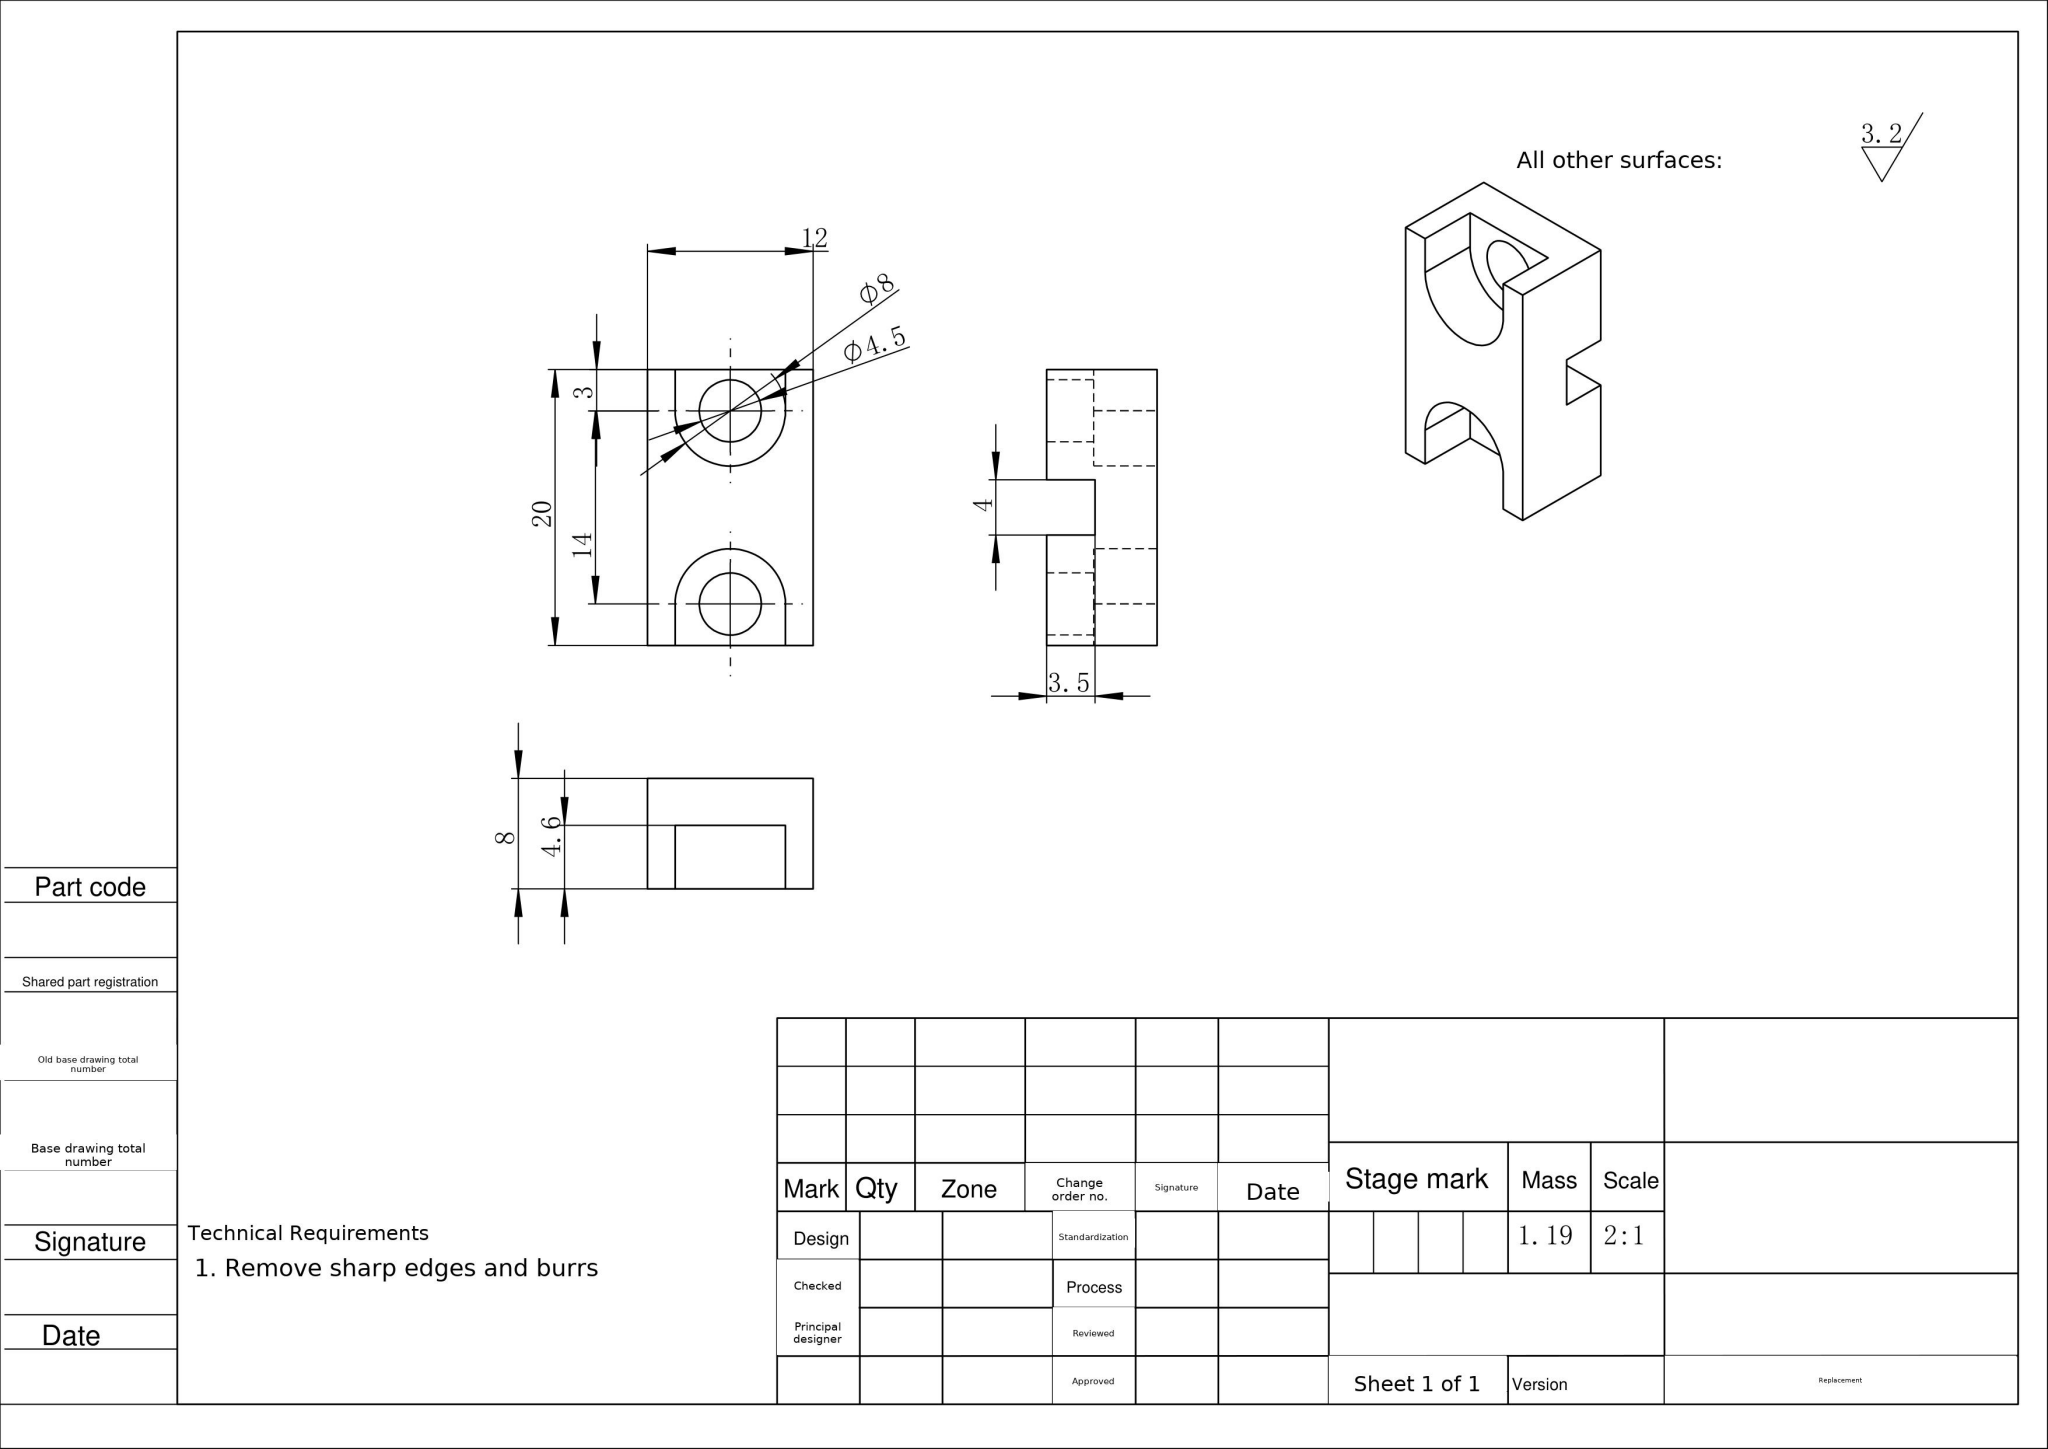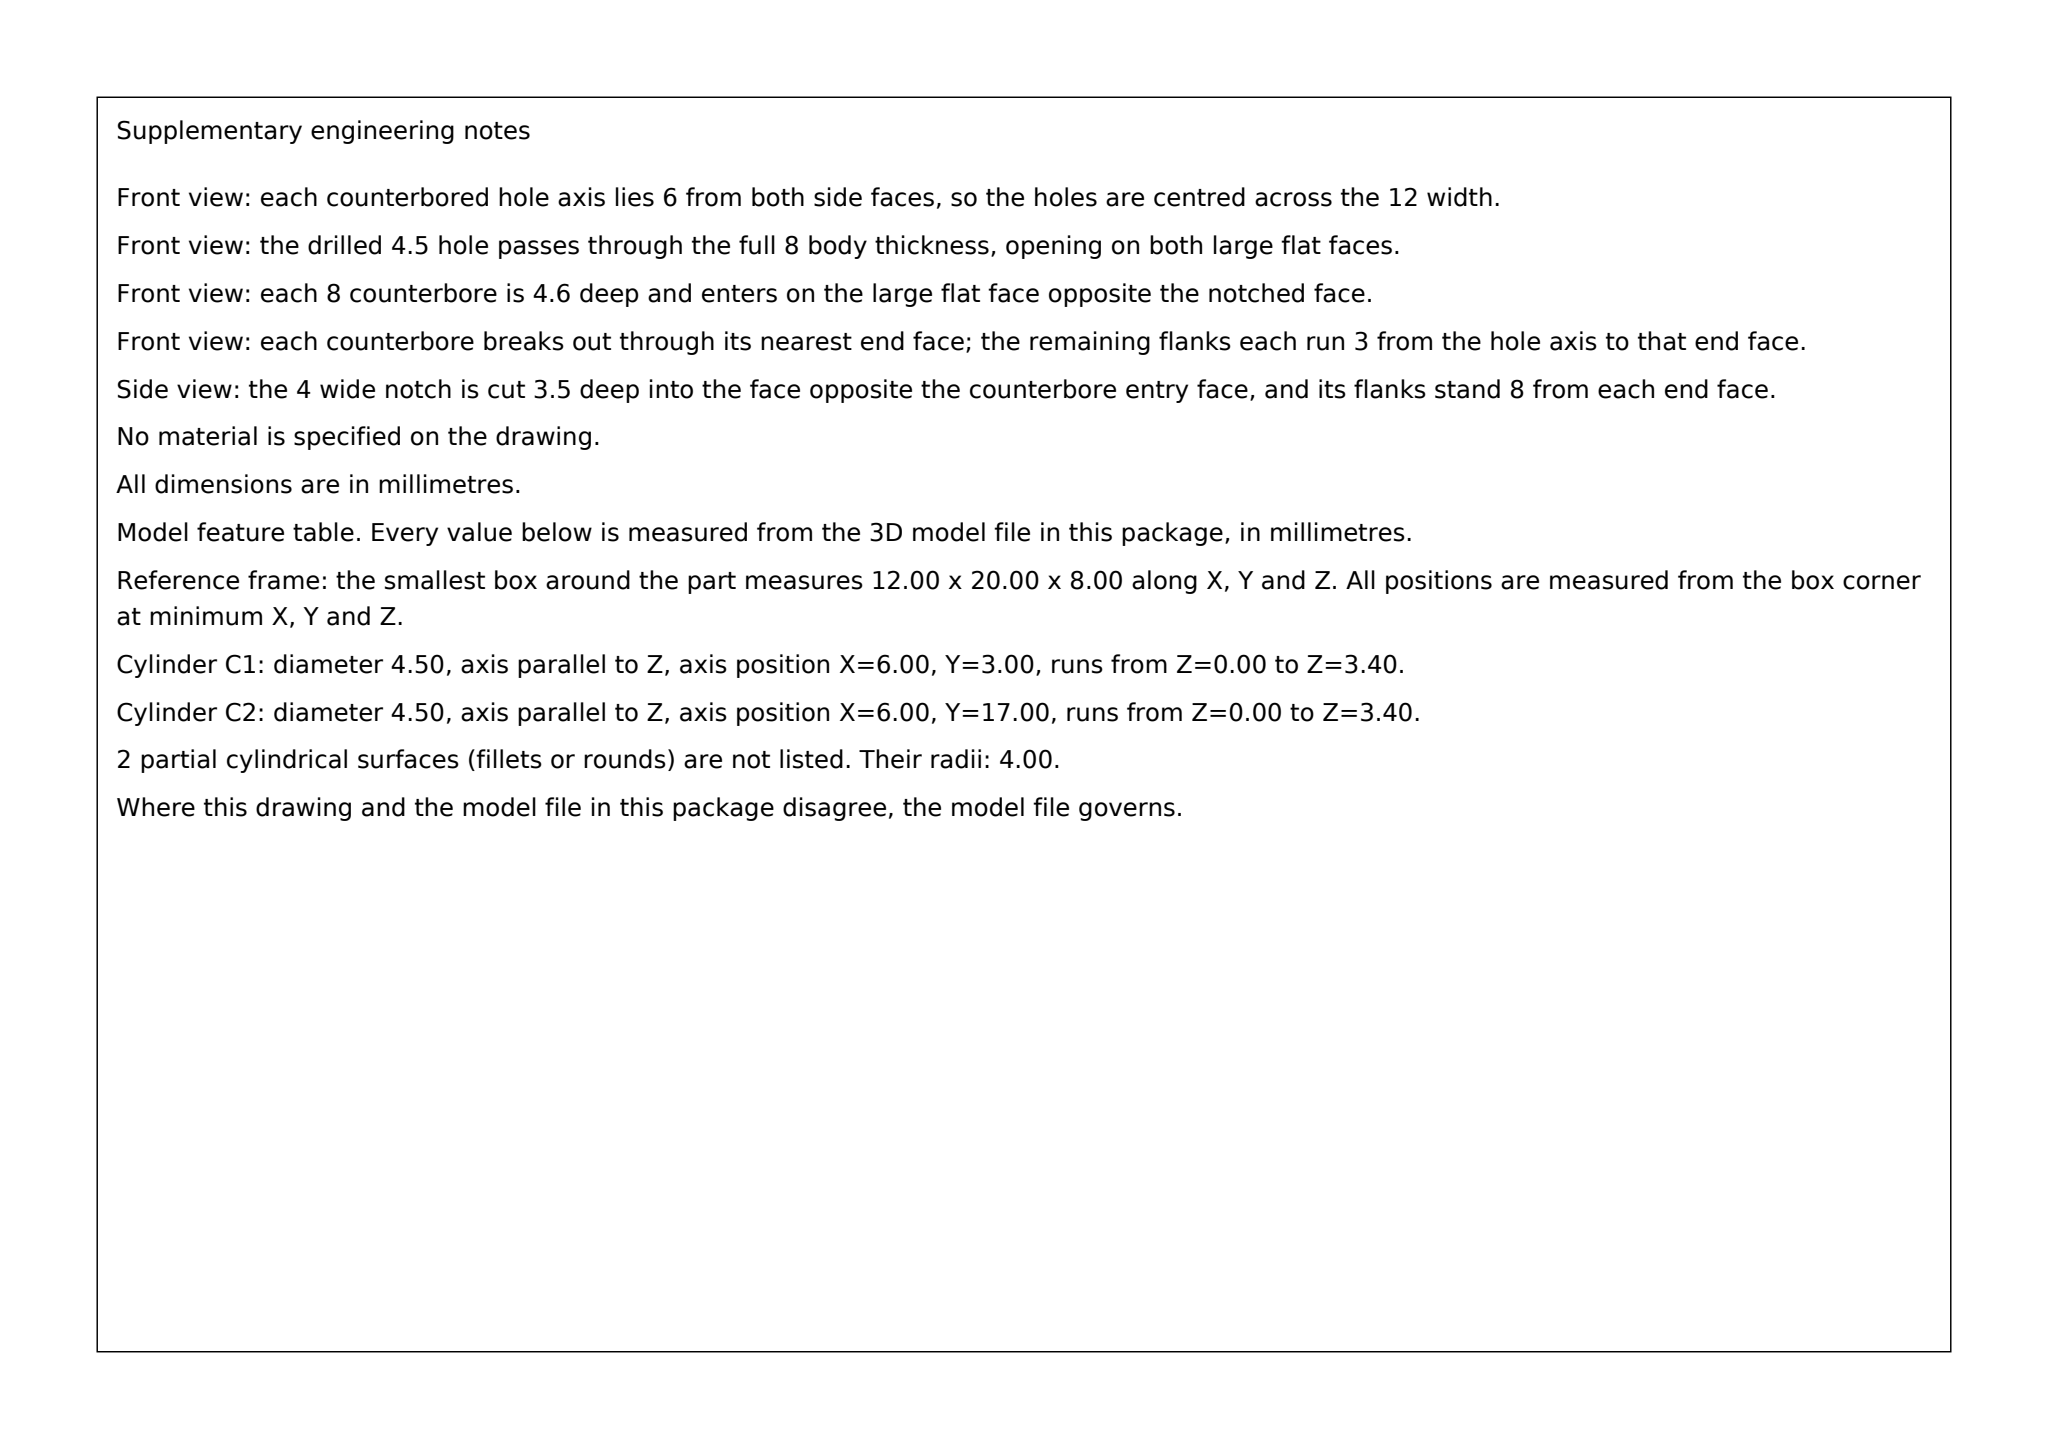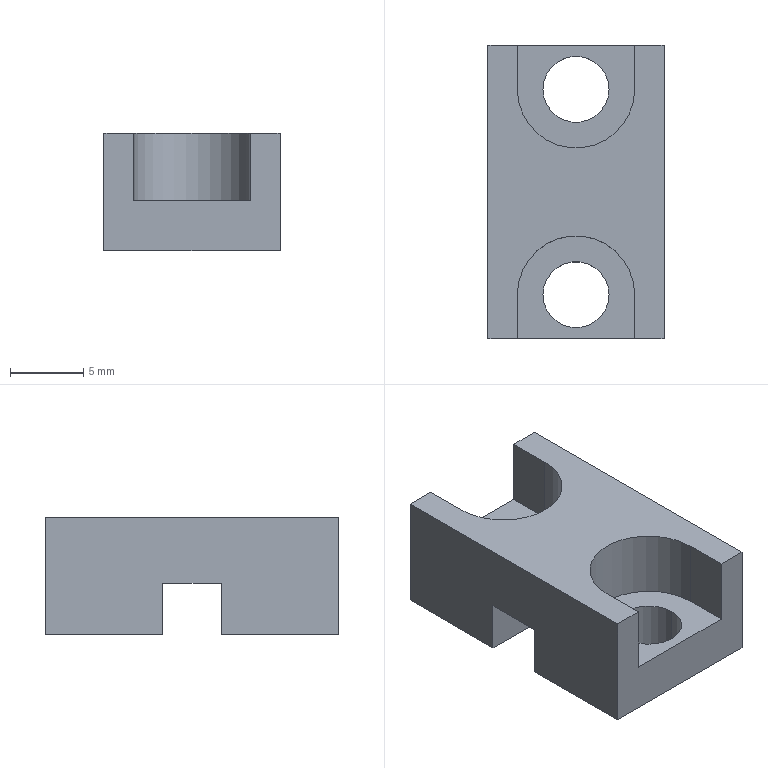Part | SolidWorks | mm | 1 solid | 22 faces | box 12 x 20 x 8 mm | volume 1192 mm3 | plane 16 | cylinder 6 | commonest cylinder face diameters 4.5 x4 8 x2
Drawing notes:
4 WIDE GROOVE SYM ABOUT 20 CL (8 FROM EACH END) | from the solid: y-planes at 8.0 and 12.0 within 0-20 bbox: 4 wide, centered on y=10
GROOVE THRU FULL 12 WIDTH, 3.5 DEEP | from the solid: groove faces span x=0 to 12 (bbox x=12); z-plane at 3.5 gives depth
build123d program:
from build123d import *

# Parameters (mm, degrees)
SKETCH1_W                                            = 12
SKETCH1_H                                            = 20
BOSS_EXTRUDE1_DEPTH                                  = 8
SKETCH2_W                                            = 12
SKETCH2_H                                            = 4
CUT_EXTRUDE1_DEPTH                                   = 3.5
HOLE_SIZE_ACCORDING_TO_TYPE_1_OF_HEXAGON_D           = 4.5
HOLE_SIZE_ACCORDING_TO_TYPE_1_OF_HEXAGON_DEPTH       = 11.5
HOLE_SIZE_ACCORDING_TO_TYPE_1_OF_HEXAGON_CBORE_D     = 8
HOLE_SIZE_ACCORDING_TO_TYPE_1_OF_HEXAGON_CBORE_DEPTH = 4.6
HOLE_SIZE_ACCORDING_TO_TYPE_1_OF_HEXAGON_TIP         = 1.352
SKETCH5_W                                            = 8
SKETCH5_H                                            = 8.409
SKETCH5_H_2                                          = 4.715
CUT_EXTRUDE2_DEPTH                                   = 4.6


with BuildPart() as part:
    # Sketch1 → Boss-Extrude1 (new body)
    with BuildSketch(Plane.XY):
        with Locations((-273.963, 122.5)):
            Rectangle(SKETCH1_W, SKETCH1_H)
    extrude(amount=BOSS_EXTRUDE1_DEPTH)

    # Sketch2 → Cut-Extrude1 (cut)
    with BuildSketch(Plane(origin=(0, 0, 0), x_dir=(-1, 0, 0), z_dir=(0, 0, -1))):
        with Locations((273.963, 122.5)):
            Rectangle(SKETCH2_W, SKETCH2_H)
    extrude(amount=-CUT_EXTRUDE1_DEPTH, mode=Mode.SUBTRACT)

    # Hole Size_According to_Type 1 of Hexagon
    with Locations(Plane.XY.offset(8)):
        with Locations((-273.963, 129.5), (-273.963, 115.5)):
            CounterBoreHole(HOLE_SIZE_ACCORDING_TO_TYPE_1_OF_HEXAGON_D / 2, HOLE_SIZE_ACCORDING_TO_TYPE_1_OF_HEXAGON_CBORE_D / 2, HOLE_SIZE_ACCORDING_TO_TYPE_1_OF_HEXAGON_CBORE_DEPTH, depth=HOLE_SIZE_ACCORDING_TO_TYPE_1_OF_HEXAGON_DEPTH)
            with Locations((0, 0, -(HOLE_SIZE_ACCORDING_TO_TYPE_1_OF_HEXAGON_DEPTH + HOLE_SIZE_ACCORDING_TO_TYPE_1_OF_HEXAGON_TIP / 2))):  # 118° drill point
                Cone(0, HOLE_SIZE_ACCORDING_TO_TYPE_1_OF_HEXAGON_D / 2, HOLE_SIZE_ACCORDING_TO_TYPE_1_OF_HEXAGON_TIP, mode=Mode.SUBTRACT)

    # Sketch5 → Cut-Extrude2 (cut)
    with BuildSketch(Plane.XY.offset(8)):
        with Locations((-273.963, 133.705)):
            Rectangle(SKETCH5_W, SKETCH5_H)
        with Locations((-273.963, 113.143)):
            Rectangle(SKETCH5_W, SKETCH5_H_2)
    extrude(amount=-CUT_EXTRUDE2_DEPTH, mode=Mode.SUBTRACT)


solid = part.part
STEP:
#1=CARTESIAN_POINT('',(-271.713,129.5,0.));
#2=VERTEX_POINT('',#1);
#3=CARTESIAN_POINT('',(-276.213,129.5,0.));
#4=VERTEX_POINT('',#3);
#5=CARTESIAN_POINT('',(-273.963,129.5,0.));
#6=DIRECTION('',(0.,0.,-1.));
#7=DIRECTION('',(-1.,0.,0.));
#8=AXIS2_PLACEMENT_3D('',#5,#6,#7);
#9=CIRCLE('',#8,2.25);
#10=EDGE_CURVE('',#2,#4,#9,.T.);
#11=ORIENTED_EDGE('',*,*,#10,.T.);
#12=CARTESIAN_POINT('',(-276.213,129.5,3.4));
#13=VERTEX_POINT('',#12);
#14=CARTESIAN_POINT('',(-276.213,129.5,8.));
#15=DIRECTION('',(0.,0.,1.));
#16=VECTOR('',#15,1000.);
#17=LINE('',#14,#16);
#18=EDGE_CURVE('',#4,#13,#17,.T.);
#19=ORIENTED_EDGE('',*,*,#18,.T.);
#20=CARTESIAN_POINT('',(-271.713,129.5,3.4));
#21=VERTEX_POINT('',#20);
#22=CARTESIAN_POINT('',(-273.963,129.5,3.4));
#23=DIRECTION('',(0.,0.,1.));
#24=DIRECTION('',(1.,0.,0.));
#25=AXIS2_PLACEMENT_3D('',#22,#23,#24);
#26=CIRCLE('',#25,2.25);
#27=EDGE_CURVE('',#13,#21,#26,.T.);
#28=ORIENTED_EDGE('',*,*,#27,.T.);
#29=CARTESIAN_POINT('',(-271.713,129.5,8.));
#30=DIRECTION('',(0.,0.,1.));
#31=VECTOR('',#30,1000.);
#32=LINE('',#29,#31);
#33=EDGE_CURVE('',#2,#21,#32,.T.);
#34=ORIENTED_EDGE('',*,*,#33,.F.);
#35=EDGE_LOOP('',(#11,#19,#28,#34));
#36=FACE_OUTER_BOUND('',#35,.T.);
#37=CARTESIAN_POINT('',(-273.963,129.5,8.));
#38=DIRECTION('',(0.,0.,1.));
#39=DIRECTION('',(1.,0.,0.));
#40=AXIS2_PLACEMENT_3D('',#37,#38,#39);
#41=CYLINDRICAL_SURFACE('',#40,2.25);
#42=ADVANCED_FACE('',(#36),#41,.F.);
#43=CARTESIAN_POINT('',(-271.713,115.5,0.));
#44=VERTEX_POINT('',#43);
#45=CARTESIAN_POINT('',(-276.213,115.5,0.));
#46=VERTEX_POINT('',#45);
#47=CARTESIAN_POINT('',(-273.963,115.5,0.));
#48=DIRECTION('',(0.,0.,-1.));
#49=DIRECTION('',(-1.,0.,0.));
#50=AXIS2_PLACEMENT_3D('',#47,#48,#49);
#51=CIRCLE('',#50,2.25);
#52=EDGE_CURVE('',#44,#46,#51,.T.);
#53=ORIENTED_EDGE('',*,*,#52,.T.);
#54=CARTESIAN_POINT('',(-276.213,115.5,3.4));
#55=VERTEX_POINT('',#54);
#56=CARTESIAN_POINT('',(-276.213,115.5,8.));
#57=DIRECTION('',(0.,0.,1.));
#58=VECTOR('',#57,1000.);
#59=LINE('',#56,#58);
#60=EDGE_CURVE('',#46,#55,#59,.T.);
#61=ORIENTED_EDGE('',*,*,#60,.T.);
#62=CARTESIAN_POINT('',(-271.713,115.5,3.4));
#63=VERTEX_POINT('',#62);
#64=CARTESIAN_POINT('',(-273.963,115.5,3.4));
#65=DIRECTION('',(0.,0.,1.));
#66=DIRECTION('',(1.,0.,0.));
#67=AXIS2_PLACEMENT_3D('',#64,#65,#66);
#68=CIRCLE('',#67,2.25);
#69=EDGE_CURVE('',#55,#63,#68,.T.);
#70=ORIENTED_EDGE('',*,*,#69,.T.);
#71=CARTESIAN_POINT('',(-271.713,115.5,8.));
#72=DIRECTION('',(0.,0.,1.));
#73=VECTOR('',#72,1000.);
#74=LINE('',#71,#73);
#75=EDGE_CURVE('',#44,#63,#74,.T.);
#76=ORIENTED_EDGE('',*,*,#75,.F.);
#77=EDGE_LOOP('',(#53,#61,#70,#76));
#78=FACE_OUTER_BOUND('',#77,.T.);
#79=CARTESIAN_POINT('',(-273.963,115.5,8.));
#80=DIRECTION('',(0.,0.,1.));
#81=DIRECTION('',(1.,0.,0.));
#82=AXIS2_PLACEMENT_3D('',#79,#80,#81);
#83=CYLINDRICAL_SURFACE('',#82,2.25);
#84=ADVANCED_FACE('',(#78),#83,.F.);
#85=CARTESIAN_POINT('',(-269.963,129.5,8.));
#86=VERTEX_POINT('',#85);
#87=CARTESIAN_POINT('',(-277.963,129.5,8.));
#88=VERTEX_POINT('',#87);
#89=CARTESIAN_POINT('',(-273.963,129.5,8.));
#90=DIRECTION('',(0.,0.,-1.));
#91=DIRECTION('',(-1.,0.,0.));
#92=AXIS2_PLACEMENT_3D('',#89,#90,#91);
#93=CIRCLE('',#92,4.);
#94=EDGE_CURVE('',#86,#88,#93,.T.);
#95=ORIENTED_EDGE('',*,*,#94,.F.);
#96=CARTESIAN_POINT('',(-269.963,129.5,3.4));
#97=VERTEX_POINT('',#96);
#98=CARTESIAN_POINT('',(-269.963,129.5,-8.207));
#99=DIRECTION('',(0.,0.,1.));
#100=VECTOR('',#99,1000.);
#101=LINE('',#98,#100);
#102=EDGE_CURVE('',#97,#86,#101,.T.);
#103=ORIENTED_EDGE('',*,*,#102,.F.);
#104=CARTESIAN_POINT('',(-277.963,129.5,3.4));
#105=VERTEX_POINT('',#104);
#106=CARTESIAN_POINT('',(-273.963,129.5,3.4));
#107=DIRECTION('',(0.,0.,1.));
#108=DIRECTION('',(1.,0.,0.));
#109=AXIS2_PLACEMENT_3D('',#106,#107,#108);
#110=CIRCLE('',#109,4.);
#111=EDGE_CURVE('',#105,#97,#110,.T.);
#112=ORIENTED_EDGE('',*,*,#111,.F.);
#113=CARTESIAN_POINT('',(-277.963,129.5,-8.207));
#114=DIRECTION('',(0.,0.,1.));
#115=VECTOR('',#114,1000.);
#116=LINE('',#113,#115);
#117=EDGE_CURVE('',#105,#88,#116,.T.);
#118=ORIENTED_EDGE('',*,*,#117,.T.);
#119=EDGE_LOOP('',(#95,#103,#112,#118));
#120=FACE_OUTER_BOUND('',#119,.T.);
#121=CARTESIAN_POINT('',(-273.963,129.5,8.));
#122=DIRECTION('',(0.,0.,1.));
#123=DIRECTION('',(1.,0.,0.));
#124=AXIS2_PLACEMENT_3D('',#121,#122,#123);
#125=CYLINDRICAL_SURFACE('',#124,4.);
#126=ADVANCED_FACE('',(#120),#125,.F.);
#127=ORIENTED_EDGE('',*,*,#52,.F.);
#128=CARTESIAN_POINT('',(-273.963,115.5,0.));
#129=DIRECTION('',(0.,0.,-1.));
#130=DIRECTION('',(-1.,0.,0.));
#131=AXIS2_PLACEMENT_3D('',#128,#129,#130);
#132=CIRCLE('',#131,2.25);
#133=EDGE_CURVE('',#46,#44,#132,.T.);
#134=ORIENTED_EDGE('',*,*,#133,.F.);
#135=EDGE_LOOP('',(#127,#134));
#136=FACE_BOUND('',#135,.T.);
#137=CARTESIAN_POINT('',(-267.963,120.5,0.));
#138=VERTEX_POINT('',#137);
#139=CARTESIAN_POINT('',(-279.963,120.5,0.));
#140=VERTEX_POINT('',#139);
#141=CARTESIAN_POINT('',(-267.963,120.5,0.));
#142=DIRECTION('',(-1.,0.,0.));
#143=VECTOR('',#142,1000.);
#144=LINE('',#141,#143);
#145=EDGE_CURVE('',#138,#140,#144,.T.);
#146=ORIENTED_EDGE('',*,*,#145,.F.);
#147=CARTESIAN_POINT('',(-267.963,112.5,0.));
#148=VERTEX_POINT('',#147);
#149=CARTESIAN_POINT('',(-267.963,132.5,0.));
#150=DIRECTION('',(0.,1.,0.));
#151=VECTOR('',#150,1000.);
#152=LINE('',#149,#151);
#153=EDGE_CURVE('',#148,#138,#152,.T.);
#154=ORIENTED_EDGE('',*,*,#153,.F.);
#155=CARTESIAN_POINT('',(-279.963,112.5,0.));
#156=VERTEX_POINT('',#155);
#157=CARTESIAN_POINT('',(-267.963,112.5,0.));
#158=DIRECTION('',(1.,0.,0.));
#159=VECTOR('',#158,1000.);
#160=LINE('',#157,#159);
#161=EDGE_CURVE('',#156,#148,#160,.T.);
#162=ORIENTED_EDGE('',*,*,#161,.F.);
#163=CARTESIAN_POINT('',(-279.963,132.5,0.));
#164=DIRECTION('',(0.,-1.,0.));
#165=VECTOR('',#164,1000.);
#166=LINE('',#163,#165);
#167=EDGE_CURVE('',#140,#156,#166,.T.);
#168=ORIENTED_EDGE('',*,*,#167,.F.);
#169=EDGE_LOOP('',(#146,#154,#162,#168));
#170=FACE_OUTER_BOUND('',#169,.T.);
#171=CARTESIAN_POINT('',(0.,0.,0.));
#172=DIRECTION('',(0.,0.,-1.));
#173=DIRECTION('',(-1.,0.,0.));
#174=AXIS2_PLACEMENT_3D('',#171,#172,#173);
#175=PLANE('',#174);
#176=ADVANCED_FACE('',(#136,#170),#175,.T.);
#177=CARTESIAN_POINT('',(-279.963,120.5,3.5));
#178=VERTEX_POINT('',#177);
#179=CARTESIAN_POINT('',(-279.963,124.5,3.5));
#180=VERTEX_POINT('',#179);
#181=CARTESIAN_POINT('',(-279.963,120.5,3.5));
#182=DIRECTION('',(0.,1.,0.));
#183=VECTOR('',#182,1000.);
#184=LINE('',#181,#183);
#185=EDGE_CURVE('',#178,#180,#184,.T.);
#186=ORIENTED_EDGE('',*,*,#185,.F.);
#187=CARTESIAN_POINT('',(-279.963,120.5,3.5));
#188=DIRECTION('',(0.,0.,-1.));
#189=VECTOR('',#188,1000.);
#190=LINE('',#187,#189);
#191=EDGE_CURVE('',#178,#140,#190,.T.);
#192=ORIENTED_EDGE('',*,*,#191,.T.);
#193=ORIENTED_EDGE('',*,*,#167,.T.);
#194=CARTESIAN_POINT('',(-279.963,112.5,8.));
#195=VERTEX_POINT('',#194);
#196=CARTESIAN_POINT('',(-279.963,112.5,8.));
#197=DIRECTION('',(0.,0.,-1.));
#198=VECTOR('',#197,1000.);
#199=LINE('',#196,#198);
#200=EDGE_CURVE('',#195,#156,#199,.T.);
#201=ORIENTED_EDGE('',*,*,#200,.F.);
#202=CARTESIAN_POINT('',(-279.963,132.5,8.));
#203=VERTEX_POINT('',#202);
#204=CARTESIAN_POINT('',(-279.963,132.5,8.));
#205=DIRECTION('',(0.,-1.,0.));
#206=VECTOR('',#205,1000.);
#207=LINE('',#204,#206);
#208=EDGE_CURVE('',#203,#195,#207,.T.);
#209=ORIENTED_EDGE('',*,*,#208,.F.);
#210=CARTESIAN_POINT('',(-279.963,132.5,0.));
#211=VERTEX_POINT('',#210);
#212=CARTESIAN_POINT('',(-279.963,132.5,8.));
#213=DIRECTION('',(0.,0.,-1.));
#214=VECTOR('',#213,1000.);
#215=LINE('',#212,#214);
#216=EDGE_CURVE('',#203,#211,#215,.T.);
#217=ORIENTED_EDGE('',*,*,#216,.T.);
#218=CARTESIAN_POINT('',(-279.963,124.5,0.));
#219=VERTEX_POINT('',#218);
#220=CARTESIAN_POINT('',(-279.963,132.5,0.));
#221=DIRECTION('',(0.,-1.,0.));
#222=VECTOR('',#221,1000.);
#223=LINE('',#220,#222);
#224=EDGE_CURVE('',#211,#219,#223,.T.);
#225=ORIENTED_EDGE('',*,*,#224,.T.);
#226=CARTESIAN_POINT('',(-279.963,124.5,3.5));
#227=DIRECTION('',(0.,0.,-1.));
#228=VECTOR('',#227,1000.);
#229=LINE('',#226,#228);
#230=EDGE_CURVE('',#180,#219,#229,.T.);
#231=ORIENTED_EDGE('',*,*,#230,.F.);
#232=EDGE_LOOP('',(#186,#192,#193,#201,#209,#217,#225,#231));
#233=FACE_OUTER_BOUND('',#232,.T.);
#234=CARTESIAN_POINT('',(-279.963,132.5,8.));
#235=DIRECTION('',(1.,0.,0.));
#236=DIRECTION('',(0.,0.,-1.));
#237=AXIS2_PLACEMENT_3D('',#234,#235,#236);
#238=PLANE('',#237);
#239=ADVANCED_FACE('',(#233),#238,.F.);
#240=CARTESIAN_POINT('',(-269.963,112.5,8.));
#241=VERTEX_POINT('',#240);
#242=CARTESIAN_POINT('',(-269.963,112.5,3.4));
#243=VERTEX_POINT('',#242);
#244=CARTESIAN_POINT('',(-269.963,112.5,8.));
#245=DIRECTION('',(0.,0.,-1.));
#246=VECTOR('',#245,1000.);
#247=LINE('',#244,#246);
#248=EDGE_CURVE('',#241,#243,#247,.T.);
#249=ORIENTED_EDGE('',*,*,#248,.T.);
#250=CARTESIAN_POINT('',(-277.963,112.5,3.4));
#251=VERTEX_POINT('',#250);
#252=CARTESIAN_POINT('',(-267.963,112.5,3.4));
#253=DIRECTION('',(-1.,0.,0.));
#254=VECTOR('',#253,1000.);
#255=LINE('',#252,#254);
#256=EDGE_CURVE('',#243,#251,#255,.T.);
#257=ORIENTED_EDGE('',*,*,#256,.T.);
#258=CARTESIAN_POINT('',(-277.963,112.5,8.));
#259=VERTEX_POINT('',#258);
#260=CARTESIAN_POINT('',(-277.963,112.5,8.));
#261=DIRECTION('',(0.,0.,1.));
#262=VECTOR('',#261,1000.);
#263=LINE('',#260,#262);
#264=EDGE_CURVE('',#251,#259,#263,.T.);
#265=ORIENTED_EDGE('',*,*,#264,.T.);
#266=CARTESIAN_POINT('',(-267.963,112.5,8.));
#267=DIRECTION('',(1.,0.,0.));
#268=VECTOR('',#267,1000.);
#269=LINE('',#266,#268);
#270=EDGE_CURVE('',#195,#259,#269,.T.);
#271=ORIENTED_EDGE('',*,*,#270,.F.);
#272=ORIENTED_EDGE('',*,*,#200,.T.);
#273=ORIENTED_EDGE('',*,*,#161,.T.);
#274=CARTESIAN_POINT('',(-267.963,112.5,8.));
#275=VERTEX_POINT('',#274);
#276=CARTESIAN_POINT('',(-267.963,112.5,8.));
#277=DIRECTION('',(0.,0.,-1.));
#278=VECTOR('',#277,1000.);
#279=LINE('',#276,#278);
#280=EDGE_CURVE('',#275,#148,#279,.T.);
#281=ORIENTED_EDGE('',*,*,#280,.F.);
#282=CARTESIAN_POINT('',(-267.963,112.5,8.));
#283=DIRECTION('',(1.,0.,0.));
#284=VECTOR('',#283,1000.);
#285=LINE('',#282,#284);
#286=EDGE_CURVE('',#241,#275,#285,.T.);
#287=ORIENTED_EDGE('',*,*,#286,.F.);
#288=EDGE_LOOP('',(#249,#257,#265,#271,#272,#273,#281,#287));
#289=FACE_OUTER_BOUND('',#288,.T.);
#290=CARTESIAN_POINT('',(-267.963,112.5,8.));
#291=DIRECTION('',(0.,1.,0.));
#292=DIRECTION('',(0.,0.,1.));
#293=AXIS2_PLACEMENT_3D('',#290,#291,#292);
#294=PLANE('',#293);
#295=ADVANCED_FACE('',(#289),#294,.F.);
#296=ORIENTED_EDGE('',*,*,#153,.T.);
#297=CARTESIAN_POINT('',(-267.963,120.5,3.5));
#298=VERTEX_POINT('',#297);
#299=CARTESIAN_POINT('',(-267.963,120.5,3.5));
#300=DIRECTION('',(0.,0.,-1.));
#301=VECTOR('',#300,1000.);
#302=LINE('',#299,#301);
#303=EDGE_CURVE('',#298,#138,#302,.T.);
#304=ORIENTED_EDGE('',*,*,#303,.F.);
#305=CARTESIAN_POINT('',(-267.963,124.5,3.5));
#306=VERTEX_POINT('',#305);
#307=CARTESIAN_POINT('',(-267.963,120.5,3.5));
#308=DIRECTION('',(0.,-1.,0.));
#309=VECTOR('',#308,1000.);
#310=LINE('',#307,#309);
#311=EDGE_CURVE('',#306,#298,#310,.T.);
#312=ORIENTED_EDGE('',*,*,#311,.F.);
#313=CARTESIAN_POINT('',(-267.963,124.5,0.));
#314=VERTEX_POINT('',#313);
#315=CARTESIAN_POINT('',(-267.963,124.5,3.5));
#316=DIRECTION('',(0.,0.,-1.));
#317=VECTOR('',#316,1000.);
#318=LINE('',#315,#317);
#319=EDGE_CURVE('',#306,#314,#318,.T.);
#320=ORIENTED_EDGE('',*,*,#319,.T.);
#321=CARTESIAN_POINT('',(-267.963,132.5,0.));
#322=VERTEX_POINT('',#321);
#323=CARTESIAN_POINT('',(-267.963,132.5,0.));
#324=DIRECTION('',(0.,1.,0.));
#325=VECTOR('',#324,1000.);
#326=LINE('',#323,#325);
#327=EDGE_CURVE('',#314,#322,#326,.T.);
#328=ORIENTED_EDGE('',*,*,#327,.T.);
#329=CARTESIAN_POINT('',(-267.963,132.5,8.));
#330=VERTEX_POINT('',#329);
#331=CARTESIAN_POINT('',(-267.963,132.5,8.));
#332=DIRECTION('',(0.,0.,-1.));
#333=VECTOR('',#332,1000.);
#334=LINE('',#331,#333);
#335=EDGE_CURVE('',#330,#322,#334,.T.);
#336=ORIENTED_EDGE('',*,*,#335,.F.);
#337=CARTESIAN_POINT('',(-267.963,132.5,8.));
#338=DIRECTION('',(0.,1.,0.));
#339=VECTOR('',#338,1000.);
#340=LINE('',#337,#339);
#341=EDGE_CURVE('',#275,#330,#340,.T.);
#342=ORIENTED_EDGE('',*,*,#341,.F.);
#343=ORIENTED_EDGE('',*,*,#280,.T.);
#344=EDGE_LOOP('',(#296,#304,#312,#320,#328,#336,#342,#343));
#345=FACE_OUTER_BOUND('',#344,.T.);
#346=CARTESIAN_POINT('',(-267.963,132.5,8.));
#347=DIRECTION('',(-1.,0.,0.));
#348=DIRECTION('',(0.,0.,1.));
#349=AXIS2_PLACEMENT_3D('',#346,#347,#348);
#350=PLANE('',#349);
#351=ADVANCED_FACE('',(#345),#350,.F.);
#352=CARTESIAN_POINT('',(-277.963,132.5,3.4));
#353=VERTEX_POINT('',#352);
#354=CARTESIAN_POINT('',(-269.963,132.5,3.4));
#355=VERTEX_POINT('',#354);
#356=CARTESIAN_POINT('',(-267.963,132.5,3.4));
#357=DIRECTION('',(1.,0.,0.));
#358=VECTOR('',#357,1000.);
#359=LINE('',#356,#358);
#360=EDGE_CURVE('',#353,#355,#359,.T.);
#361=ORIENTED_EDGE('',*,*,#360,.T.);
#362=CARTESIAN_POINT('',(-269.963,132.5,8.));
#363=VERTEX_POINT('',#362);
#364=CARTESIAN_POINT('',(-269.963,132.5,8.));
#365=DIRECTION('',(0.,0.,1.));
#366=VECTOR('',#365,1000.);
#367=LINE('',#364,#366);
#368=EDGE_CURVE('',#355,#363,#367,.T.);
#369=ORIENTED_EDGE('',*,*,#368,.T.);
#370=CARTESIAN_POINT('',(-267.963,132.5,8.));
#371=DIRECTION('',(-1.,0.,0.));
#372=VECTOR('',#371,1000.);
#373=LINE('',#370,#372);
#374=EDGE_CURVE('',#330,#363,#373,.T.);
#375=ORIENTED_EDGE('',*,*,#374,.F.);
#376=ORIENTED_EDGE('',*,*,#335,.T.);
#377=CARTESIAN_POINT('',(-267.963,132.5,0.));
#378=DIRECTION('',(-1.,0.,0.));
#379=VECTOR('',#378,1000.);
#380=LINE('',#377,#379);
#381=EDGE_CURVE('',#322,#211,#380,.T.);
#382=ORIENTED_EDGE('',*,*,#381,.T.);
#383=ORIENTED_EDGE('',*,*,#216,.F.);
#384=CARTESIAN_POINT('',(-277.963,132.5,8.));
#385=VERTEX_POINT('',#384);
#386=CARTESIAN_POINT('',(-267.963,132.5,8.));
#387=DIRECTION('',(-1.,0.,0.));
#388=VECTOR('',#387,1000.);
#389=LINE('',#386,#388);
#390=EDGE_CURVE('',#385,#203,#389,.T.);
#391=ORIENTED_EDGE('',*,*,#390,.F.);
#392=CARTESIAN_POINT('',(-277.963,132.5,8.));
#393=DIRECTION('',(0.,0.,-1.));
#394=VECTOR('',#393,1000.);
#395=LINE('',#392,#394);
#396=EDGE_CURVE('',#385,#353,#395,.T.);
#397=ORIENTED_EDGE('',*,*,#396,.T.);
#398=EDGE_LOOP('',(#361,#369,#375,#376,#382,#383,#391,#397));
#399=FACE_OUTER_BOUND('',#398,.T.);
#400=CARTESIAN_POINT('',(-267.963,132.5,8.));
#401=DIRECTION('',(0.,-1.,0.));
#402=DIRECTION('',(0.,0.,-1.));
#403=AXIS2_PLACEMENT_3D('',#400,#401,#402);
#404=PLANE('',#403);
#405=ADVANCED_FACE('',(#399),#404,.F.);
#406=ORIENTED_EDGE('',*,*,#374,.T.);
#407=CARTESIAN_POINT('',(-269.963,129.5,8.));
#408=DIRECTION('',(0.,1.,0.));
#409=VECTOR('',#408,1000.);
#410=LINE('',#407,#409);
#411=EDGE_CURVE('',#86,#363,#410,.T.);
#412=ORIENTED_EDGE('',*,*,#411,.F.);
#413=ORIENTED_EDGE('',*,*,#94,.T.);
#414=CARTESIAN_POINT('',(-277.963,129.5,8.));
#415=DIRECTION('',(0.,-1.,0.));
#416=VECTOR('',#415,1000.);
#417=LINE('',#414,#416);
#418=EDGE_CURVE('',#385,#88,#417,.T.);
#419=ORIENTED_EDGE('',*,*,#418,.F.);
#420=ORIENTED_EDGE('',*,*,#390,.T.);
#421=ORIENTED_EDGE('',*,*,#208,.T.);
#422=ORIENTED_EDGE('',*,*,#270,.T.);
#423=CARTESIAN_POINT('',(-277.963,115.5,8.));
#424=VERTEX_POINT('',#423);
#425=CARTESIAN_POINT('',(-277.963,115.5,8.));
#426=DIRECTION('',(0.,-1.,0.));
#427=VECTOR('',#426,1000.);
#428=LINE('',#425,#427);
#429=EDGE_CURVE('',#424,#259,#428,.T.);
#430=ORIENTED_EDGE('',*,*,#429,.F.);
#431=CARTESIAN_POINT('',(-269.963,115.5,8.));
#432=VERTEX_POINT('',#431);
#433=CARTESIAN_POINT('',(-273.963,115.5,8.));
#434=DIRECTION('',(0.,0.,1.));
#435=DIRECTION('',(1.,0.,0.));
#436=AXIS2_PLACEMENT_3D('',#433,#434,#435);
#437=CIRCLE('',#436,4.);
#438=EDGE_CURVE('',#432,#424,#437,.T.);
#439=ORIENTED_EDGE('',*,*,#438,.F.);
#440=CARTESIAN_POINT('',(-269.963,115.5,8.));
#441=DIRECTION('',(0.,1.,0.));
#442=VECTOR('',#441,1000.);
#443=LINE('',#440,#442);
#444=EDGE_CURVE('',#241,#432,#443,.T.);
#445=ORIENTED_EDGE('',*,*,#444,.F.);
#446=ORIENTED_EDGE('',*,*,#286,.T.);
#447=ORIENTED_EDGE('',*,*,#341,.T.);
#448=EDGE_LOOP('',(#406,#412,#413,#419,#420,#421,#422,#430,#439,#445,#446,#447));
#449=FACE_OUTER_BOUND('',#448,.T.);
#450=CARTESIAN_POINT('',(0.,0.,8.));
#451=DIRECTION('',(0.,0.,-1.));
#452=DIRECTION('',(-1.,0.,0.));
#453=AXIS2_PLACEMENT_3D('',#450,#451,#452);
#454=PLANE('',#453);
#455=ADVANCED_FACE('',(#449),#454,.F.);
#456=ORIENTED_EDGE('',*,*,#10,.F.);
#457=CARTESIAN_POINT('',(-273.963,129.5,0.));
#458=DIRECTION('',(0.,0.,-1.));
#459=DIRECTION('',(-1.,0.,0.));
#460=AXIS2_PLACEMENT_3D('',#457,#458,#459);
#461=CIRCLE('',#460,2.25);
#462=EDGE_CURVE('',#4,#2,#461,.T.);
#463=ORIENTED_EDGE('',*,*,#462,.F.);
#464=EDGE_LOOP('',(#456,#463));
#465=FACE_BOUND('',#464,.T.);
#466=CARTESIAN_POINT('',(-267.963,124.5,0.));
#467=DIRECTION('',(1.,0.,0.));
#468=VECTOR('',#467,1000.);
#469=LINE('',#466,#468);
#470=EDGE_CURVE('',#219,#314,#469,.T.);
#471=ORIENTED_EDGE('',*,*,#470,.F.);
#472=ORIENTED_EDGE('',*,*,#224,.F.);
#473=ORIENTED_EDGE('',*,*,#381,.F.);
#474=ORIENTED_EDGE('',*,*,#327,.F.);
#475=EDGE_LOOP('',(#471,#472,#473,#474));
#476=FACE_OUTER_BOUND('',#475,.T.);
#477=CARTESIAN_POINT('',(0.,0.,0.));
#478=DIRECTION('',(0.,0.,-1.));
#479=DIRECTION('',(-1.,0.,0.));
#480=AXIS2_PLACEMENT_3D('',#477,#478,#479);
#481=PLANE('',#480);
#482=ADVANCED_FACE('',(#465,#476),#481,.T.);
#483=ORIENTED_EDGE('',*,*,#145,.T.);
#484=ORIENTED_EDGE('',*,*,#191,.F.);
#485=CARTESIAN_POINT('',(-267.963,120.5,3.5));
#486=DIRECTION('',(-1.,0.,0.));
#487=VECTOR('',#486,1000.);
#488=LINE('',#485,#487);
#489=EDGE_CURVE('',#298,#178,#488,.T.);
#490=ORIENTED_EDGE('',*,*,#489,.F.);
#491=ORIENTED_EDGE('',*,*,#303,.T.);
#492=EDGE_LOOP('',(#483,#484,#490,#491));
#493=FACE_OUTER_BOUND('',#492,.T.);
#494=CARTESIAN_POINT('',(-267.963,120.5,3.5));
#495=DIRECTION('',(0.,-1.,0.));
#496=DIRECTION('',(0.,0.,-1.));
#497=AXIS2_PLACEMENT_3D('',#494,#495,#496);
#498=PLANE('',#497);
#499=ADVANCED_FACE('',(#493),#498,.F.);
#500=ORIENTED_EDGE('',*,*,#470,.T.);
#501=ORIENTED_EDGE('',*,*,#319,.F.);
#502=CARTESIAN_POINT('',(-267.963,124.5,3.5));
#503=DIRECTION('',(1.,0.,0.));
#504=VECTOR('',#503,1000.);
#505=LINE('',#502,#504);
#506=EDGE_CURVE('',#180,#306,#505,.T.);
#507=ORIENTED_EDGE('',*,*,#506,.F.);
#508=ORIENTED_EDGE('',*,*,#230,.T.);
#509=EDGE_LOOP('',(#500,#501,#507,#508));
#510=FACE_OUTER_BOUND('',#509,.T.);
#511=CARTESIAN_POINT('',(-267.963,124.5,3.5));
#512=DIRECTION('',(0.,1.,0.));
#513=DIRECTION('',(0.,0.,1.));
#514=AXIS2_PLACEMENT_3D('',#511,#512,#513);
#515=PLANE('',#514);
#516=ADVANCED_FACE('',(#510),#515,.F.);
#517=ORIENTED_EDGE('',*,*,#185,.T.);
#518=ORIENTED_EDGE('',*,*,#506,.T.);
#519=ORIENTED_EDGE('',*,*,#311,.T.);
#520=ORIENTED_EDGE('',*,*,#489,.T.);
#521=EDGE_LOOP('',(#517,#518,#519,#520));
#522=FACE_OUTER_BOUND('',#521,.T.);
#523=CARTESIAN_POINT('',(0.,0.,3.5));
#524=DIRECTION('',(0.,0.,1.));
#525=DIRECTION('',(1.,0.,0.));
#526=AXIS2_PLACEMENT_3D('',#523,#524,#525);
#527=PLANE('',#526);
#528=ADVANCED_FACE('',(#522),#527,.F.);
#529=CARTESIAN_POINT('',(-273.963,115.5,3.4));
#530=DIRECTION('',(0.,0.,1.));
#531=DIRECTION('',(1.,0.,0.));
#532=AXIS2_PLACEMENT_3D('',#529,#530,#531);
#533=CIRCLE('',#532,2.25);
#534=EDGE_CURVE('',#63,#55,#533,.T.);
#535=ORIENTED_EDGE('',*,*,#534,.F.);
#536=ORIENTED_EDGE('',*,*,#69,.F.);
#537=EDGE_LOOP('',(#535,#536));
#538=FACE_BOUND('',#537,.T.);
#539=CARTESIAN_POINT('',(-269.963,115.5,3.4));
#540=VERTEX_POINT('',#539);
#541=CARTESIAN_POINT('',(-277.963,115.5,3.4));
#542=VERTEX_POINT('',#541);
#543=CARTESIAN_POINT('',(-273.963,115.5,3.4));
#544=DIRECTION('',(0.,0.,1.));
#545=DIRECTION('',(1.,0.,0.));
#546=AXIS2_PLACEMENT_3D('',#543,#544,#545);
#547=CIRCLE('',#546,4.);
#548=EDGE_CURVE('',#540,#542,#547,.T.);
#549=ORIENTED_EDGE('',*,*,#548,.T.);
#550=CARTESIAN_POINT('',(-277.963,115.5,3.4));
#551=DIRECTION('',(0.,-1.,0.));
#552=VECTOR('',#551,1000.);
#553=LINE('',#550,#552);
#554=EDGE_CURVE('',#542,#251,#553,.T.);
#555=ORIENTED_EDGE('',*,*,#554,.T.);
#556=ORIENTED_EDGE('',*,*,#256,.F.);
#557=CARTESIAN_POINT('',(-269.963,115.5,3.4));
#558=DIRECTION('',(0.,1.,0.));
#559=VECTOR('',#558,1000.);
#560=LINE('',#557,#559);
#561=EDGE_CURVE('',#243,#540,#560,.T.);
#562=ORIENTED_EDGE('',*,*,#561,.T.);
#563=EDGE_LOOP('',(#549,#555,#556,#562));
#564=FACE_OUTER_BOUND('',#563,.T.);
#565=CARTESIAN_POINT('',(-271.713,115.5,3.4));
#566=DIRECTION('',(0.,0.,-1.));
#567=DIRECTION('',(-1.,0.,0.));
#568=AXIS2_PLACEMENT_3D('',#565,#566,#567);
#569=PLANE('',#568);
#570=ADVANCED_FACE('',(#538,#564),#569,.F.);
#571=ORIENTED_EDGE('',*,*,#548,.F.);
#572=CARTESIAN_POINT('',(-269.963,115.5,-8.207));
#573=DIRECTION('',(0.,0.,1.));
#574=VECTOR('',#573,1000.);
#575=LINE('',#572,#574);
#576=EDGE_CURVE('',#540,#432,#575,.T.);
#577=ORIENTED_EDGE('',*,*,#576,.T.);
#578=ORIENTED_EDGE('',*,*,#438,.T.);
#579=CARTESIAN_POINT('',(-277.963,115.5,-8.207));
#580=DIRECTION('',(0.,0.,1.));
#581=VECTOR('',#580,1000.);
#582=LINE('',#579,#581);
#583=EDGE_CURVE('',#542,#424,#582,.T.);
#584=ORIENTED_EDGE('',*,*,#583,.F.);
#585=EDGE_LOOP('',(#571,#577,#578,#584));
#586=FACE_OUTER_BOUND('',#585,.T.);
#587=CARTESIAN_POINT('',(-273.963,115.5,8.));
#588=DIRECTION('',(0.,0.,1.));
#589=DIRECTION('',(1.,0.,0.));
#590=AXIS2_PLACEMENT_3D('',#587,#588,#589);
#591=CYLINDRICAL_SURFACE('',#590,4.);
#592=ADVANCED_FACE('',(#586),#591,.F.);
#593=ORIENTED_EDGE('',*,*,#60,.F.);
#594=ORIENTED_EDGE('',*,*,#133,.T.);
#595=ORIENTED_EDGE('',*,*,#75,.T.);
#596=ORIENTED_EDGE('',*,*,#534,.T.);
#597=EDGE_LOOP('',(#593,#594,#595,#596));
#598=FACE_OUTER_BOUND('',#597,.T.);
#599=CARTESIAN_POINT('',(-273.963,115.5,8.));
#600=DIRECTION('',(0.,0.,1.));
#601=DIRECTION('',(1.,0.,0.));
#602=AXIS2_PLACEMENT_3D('',#599,#600,#601);
#603=CYLINDRICAL_SURFACE('',#602,2.25);
#604=ADVANCED_FACE('',(#598),#603,.F.);
#605=CARTESIAN_POINT('',(-273.963,129.5,3.4));
#606=DIRECTION('',(0.,0.,1.));
#607=DIRECTION('',(1.,0.,0.));
#608=AXIS2_PLACEMENT_3D('',#605,#606,#607);
#609=CIRCLE('',#608,2.25);
#610=EDGE_CURVE('',#21,#13,#609,.T.);
#611=ORIENTED_EDGE('',*,*,#610,.F.);
#612=ORIENTED_EDGE('',*,*,#27,.F.);
#613=EDGE_LOOP('',(#611,#612));
#614=FACE_BOUND('',#613,.T.);
#615=ORIENTED_EDGE('',*,*,#111,.T.);
#616=CARTESIAN_POINT('',(-269.963,129.5,3.4));
#617=DIRECTION('',(0.,1.,0.));
#618=VECTOR('',#617,1000.);
#619=LINE('',#616,#618);
#620=EDGE_CURVE('',#97,#355,#619,.T.);
#621=ORIENTED_EDGE('',*,*,#620,.T.);
#622=ORIENTED_EDGE('',*,*,#360,.F.);
#623=CARTESIAN_POINT('',(-277.963,129.5,3.4));
#624=DIRECTION('',(0.,-1.,0.));
#625=VECTOR('',#624,1000.);
#626=LINE('',#623,#625);
#627=EDGE_CURVE('',#353,#105,#626,.T.);
#628=ORIENTED_EDGE('',*,*,#627,.T.);
#629=EDGE_LOOP('',(#615,#621,#622,#628));
#630=FACE_OUTER_BOUND('',#629,.T.);
#631=CARTESIAN_POINT('',(-271.713,129.5,3.4));
#632=DIRECTION('',(0.,0.,-1.));
#633=DIRECTION('',(-1.,0.,0.));
#634=AXIS2_PLACEMENT_3D('',#631,#632,#633);
#635=PLANE('',#634);
#636=ADVANCED_FACE('',(#614,#630),#635,.F.);
#637=ORIENTED_EDGE('',*,*,#18,.F.);
#638=ORIENTED_EDGE('',*,*,#462,.T.);
#639=ORIENTED_EDGE('',*,*,#33,.T.);
#640=ORIENTED_EDGE('',*,*,#610,.T.);
#641=EDGE_LOOP('',(#637,#638,#639,#640));
#642=FACE_OUTER_BOUND('',#641,.T.);
#643=CARTESIAN_POINT('',(-273.963,129.5,8.));
#644=DIRECTION('',(0.,0.,1.));
#645=DIRECTION('',(1.,0.,0.));
#646=AXIS2_PLACEMENT_3D('',#643,#644,#645);
#647=CYLINDRICAL_SURFACE('',#646,2.25);
#648=ADVANCED_FACE('',(#642),#647,.F.);
#649=ORIENTED_EDGE('',*,*,#418,.T.);
#650=ORIENTED_EDGE('',*,*,#117,.F.);
#651=ORIENTED_EDGE('',*,*,#627,.F.);
#652=ORIENTED_EDGE('',*,*,#396,.F.);
#653=EDGE_LOOP('',(#649,#650,#651,#652));
#654=FACE_OUTER_BOUND('',#653,.T.);
#655=CARTESIAN_POINT('',(-277.963,129.5,-8.207));
#656=DIRECTION('',(-1.,0.,0.));
#657=DIRECTION('',(0.,0.,1.));
#658=AXIS2_PLACEMENT_3D('',#655,#656,#657);
#659=PLANE('',#658);
#660=ADVANCED_FACE('',(#654),#659,.F.);
#661=ORIENTED_EDGE('',*,*,#620,.F.);
#662=ORIENTED_EDGE('',*,*,#102,.T.);
#663=ORIENTED_EDGE('',*,*,#411,.T.);
#664=ORIENTED_EDGE('',*,*,#368,.F.);
#665=EDGE_LOOP('',(#661,#662,#663,#664));
#666=FACE_OUTER_BOUND('',#665,.T.);
#667=CARTESIAN_POINT('',(-269.963,129.5,-8.207));
#668=DIRECTION('',(1.,0.,0.));
#669=DIRECTION('',(0.,0.,-1.));
#670=AXIS2_PLACEMENT_3D('',#667,#668,#669);
#671=PLANE('',#670);
#672=ADVANCED_FACE('',(#666),#671,.F.);
#673=ORIENTED_EDGE('',*,*,#554,.F.);
#674=ORIENTED_EDGE('',*,*,#583,.T.);
#675=ORIENTED_EDGE('',*,*,#429,.T.);
#676=ORIENTED_EDGE('',*,*,#264,.F.);
#677=EDGE_LOOP('',(#673,#674,#675,#676));
#678=FACE_OUTER_BOUND('',#677,.T.);
#679=CARTESIAN_POINT('',(-277.963,115.5,-8.207));
#680=DIRECTION('',(-1.,0.,0.));
#681=DIRECTION('',(0.,0.,1.));
#682=AXIS2_PLACEMENT_3D('',#679,#680,#681);
#683=PLANE('',#682);
#684=ADVANCED_FACE('',(#678),#683,.F.);
#685=ORIENTED_EDGE('',*,*,#444,.T.);
#686=ORIENTED_EDGE('',*,*,#576,.F.);
#687=ORIENTED_EDGE('',*,*,#561,.F.);
#688=ORIENTED_EDGE('',*,*,#248,.F.);
#689=EDGE_LOOP('',(#685,#686,#687,#688));
#690=FACE_OUTER_BOUND('',#689,.T.);
#691=CARTESIAN_POINT('',(-269.963,115.5,-8.207));
#692=DIRECTION('',(1.,0.,0.));
#693=DIRECTION('',(0.,0.,-1.));
#694=AXIS2_PLACEMENT_3D('',#691,#692,#693);
#695=PLANE('',#694);
#696=ADVANCED_FACE('',(#690),#695,.F.);
#697=CLOSED_SHELL('',(#42,#84,#126,#176,#239,#295,#351,#405,#455,#482,#499,#516,#528,#570,#592,#604,#636,#648,#660,#672,#684,#696));
#698=MANIFOLD_SOLID_BREP('',#697);
#699=CARTESIAN_POINT('',(0.,0.,0.));
#700=DIRECTION('',(0.,0.,1.));
#701=DIRECTION('',(1.,0.,0.));
#702=AXIS2_PLACEMENT_3D('',#699,#700,#701);
#703=(LENGTH_UNIT()NAMED_UNIT(*)SI_UNIT(.MILLI.,.METRE.));
#704=UNCERTAINTY_MEASURE_WITH_UNIT(LENGTH_MEASURE(0.00001),#703,'','');
#705=(NAMED_UNIT(*)PLANE_ANGLE_UNIT()SI_UNIT($,.RADIAN.));
#706=(NAMED_UNIT(*)SI_UNIT($,.STERADIAN.)SOLID_ANGLE_UNIT());
#707=(GEOMETRIC_REPRESENTATION_CONTEXT(3)GLOBAL_UNCERTAINTY_ASSIGNED_CONTEXT((#704))GLOBAL_UNIT_ASSIGNED_CONTEXT((#703,#705,#706))REPRESENTATION_CONTEXT('',''));
#708=ADVANCED_BREP_SHAPE_REPRESENTATION('',(#698,#702),#707);